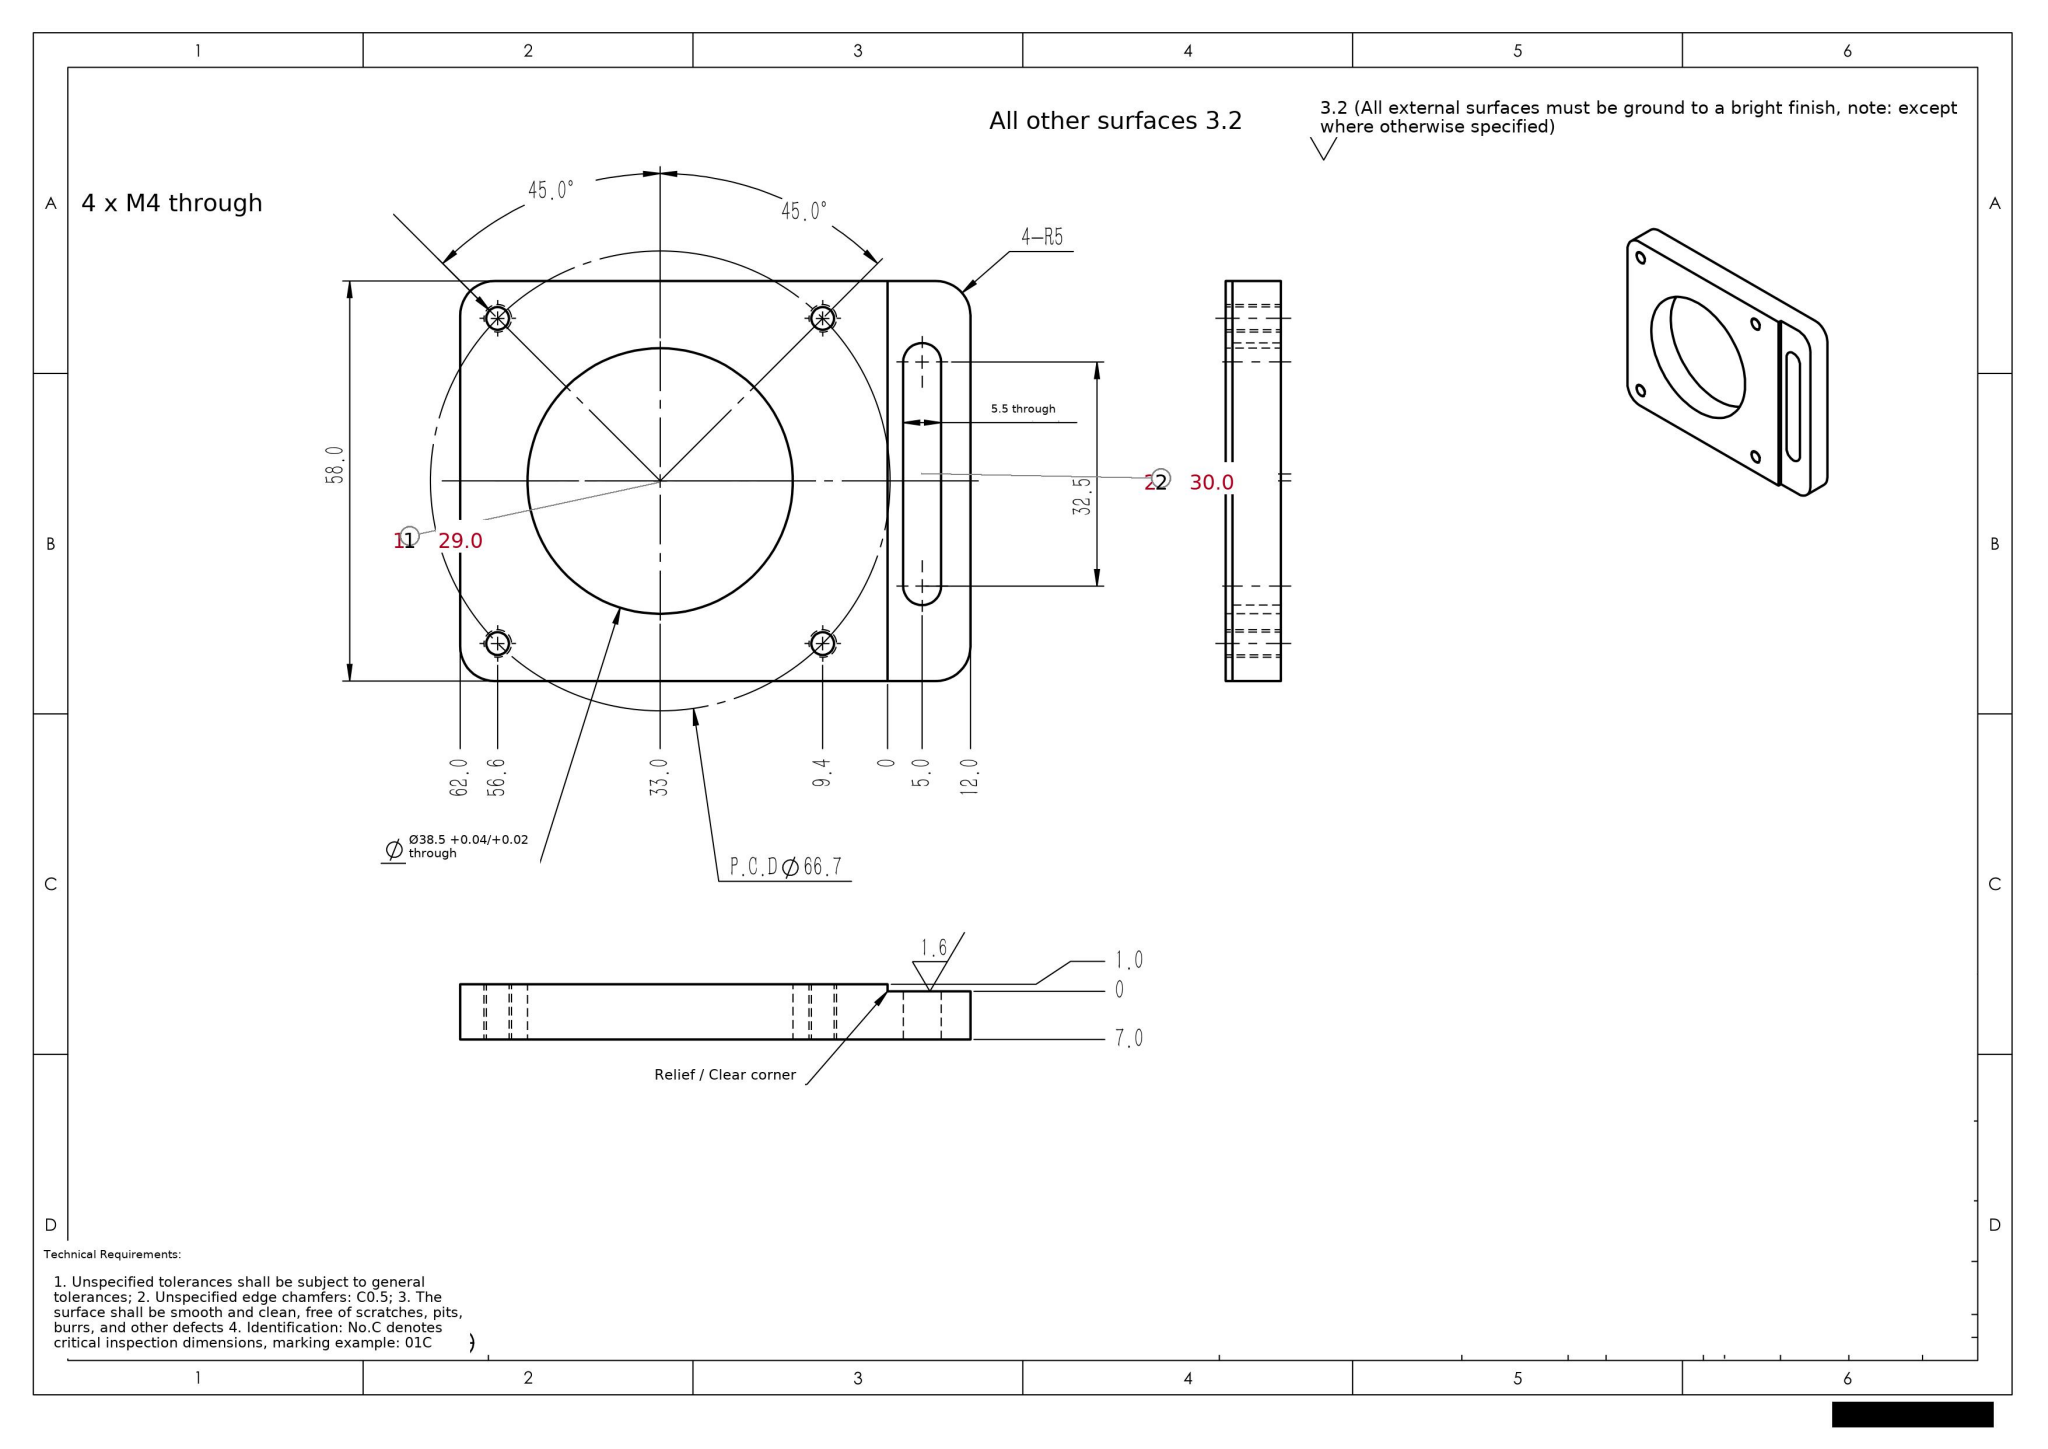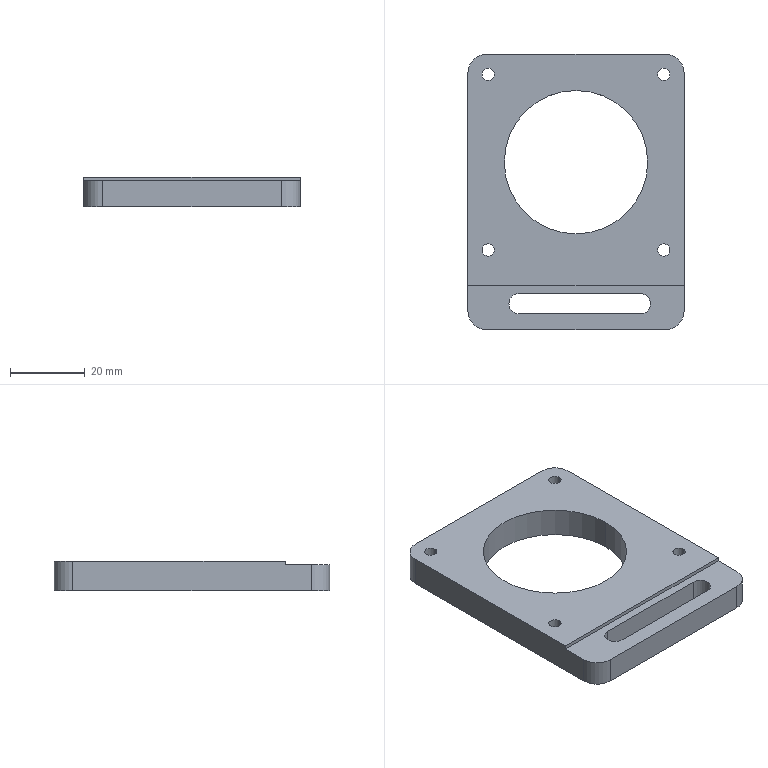Part | SolidWorks | mm | 1 solid | 27 faces | box 58 x 74 x 8 mm | volume 22475 mm3 | cylinder 17 | plane 10 | commonest cylinder face diameters 3.3 x8 10 x4 5.5 x3 38.5 x2
STEP:
#1=CARTESIAN_POINT('',(21.92,-15.57,0.));
#2=VERTEX_POINT('',#1);
#3=CARTESIAN_POINT('',(25.22,-15.57,0.));
#4=VERTEX_POINT('',#3);
#5=CARTESIAN_POINT('',(23.57,-15.57,0.));
#6=DIRECTION('',(0.,0.,1.));
#7=DIRECTION('',(1.,0.,0.));
#8=AXIS2_PLACEMENT_3D('',#5,#6,#7);
#9=CIRCLE('',#8,1.65);
#10=EDGE_CURVE('',#2,#4,#9,.T.);
#11=ORIENTED_EDGE('',*,*,#10,.F.);
#12=CARTESIAN_POINT('',(21.92,-15.57,8.));
#13=VERTEX_POINT('',#12);
#14=CARTESIAN_POINT('',(21.92,-15.57,8.));
#15=DIRECTION('',(0.,0.,1.));
#16=VECTOR('',#15,1000.);
#17=LINE('',#14,#16);
#18=EDGE_CURVE('',#2,#13,#17,.T.);
#19=ORIENTED_EDGE('',*,*,#18,.T.);
#20=CARTESIAN_POINT('',(25.22,-15.57,8.));
#21=VERTEX_POINT('',#20);
#22=CARTESIAN_POINT('',(23.57,-15.57,8.));
#23=DIRECTION('',(0.,0.,1.));
#24=DIRECTION('',(1.,0.,0.));
#25=AXIS2_PLACEMENT_3D('',#22,#23,#24);
#26=CIRCLE('',#25,1.65);
#27=EDGE_CURVE('',#13,#21,#26,.T.);
#28=ORIENTED_EDGE('',*,*,#27,.T.);
#29=CARTESIAN_POINT('',(25.22,-15.57,8.));
#30=DIRECTION('',(0.,0.,1.));
#31=VECTOR('',#30,1000.);
#32=LINE('',#29,#31);
#33=EDGE_CURVE('',#4,#21,#32,.T.);
#34=ORIENTED_EDGE('',*,*,#33,.F.);
#35=EDGE_LOOP('',(#11,#19,#28,#34));
#36=FACE_OUTER_BOUND('',#35,.T.);
#37=CARTESIAN_POINT('',(23.57,-15.57,8.));
#38=DIRECTION('',(0.,0.,1.));
#39=DIRECTION('',(1.,0.,0.));
#40=AXIS2_PLACEMENT_3D('',#37,#38,#39);
#41=CYLINDRICAL_SURFACE('',#40,1.65);
#42=ADVANCED_FACE('',(#36),#41,.F.);
#43=CARTESIAN_POINT('',(-25.22,-15.57,0.));
#44=VERTEX_POINT('',#43);
#45=CARTESIAN_POINT('',(-21.92,-15.57,0.));
#46=VERTEX_POINT('',#45);
#47=CARTESIAN_POINT('',(-23.57,-15.57,0.));
#48=DIRECTION('',(0.,0.,1.));
#49=DIRECTION('',(1.,0.,0.));
#50=AXIS2_PLACEMENT_3D('',#47,#48,#49);
#51=CIRCLE('',#50,1.65);
#52=EDGE_CURVE('',#44,#46,#51,.T.);
#53=ORIENTED_EDGE('',*,*,#52,.F.);
#54=CARTESIAN_POINT('',(-25.22,-15.57,8.));
#55=VERTEX_POINT('',#54);
#56=CARTESIAN_POINT('',(-25.22,-15.57,8.));
#57=DIRECTION('',(0.,0.,1.));
#58=VECTOR('',#57,1000.);
#59=LINE('',#56,#58);
#60=EDGE_CURVE('',#44,#55,#59,.T.);
#61=ORIENTED_EDGE('',*,*,#60,.T.);
#62=CARTESIAN_POINT('',(-21.92,-15.57,8.));
#63=VERTEX_POINT('',#62);
#64=CARTESIAN_POINT('',(-23.57,-15.57,8.));
#65=DIRECTION('',(0.,0.,1.));
#66=DIRECTION('',(1.,0.,0.));
#67=AXIS2_PLACEMENT_3D('',#64,#65,#66);
#68=CIRCLE('',#67,1.65);
#69=EDGE_CURVE('',#55,#63,#68,.T.);
#70=ORIENTED_EDGE('',*,*,#69,.T.);
#71=CARTESIAN_POINT('',(-21.92,-15.57,8.));
#72=DIRECTION('',(0.,0.,1.));
#73=VECTOR('',#72,1000.);
#74=LINE('',#71,#73);
#75=EDGE_CURVE('',#46,#63,#74,.T.);
#76=ORIENTED_EDGE('',*,*,#75,.F.);
#77=EDGE_LOOP('',(#53,#61,#70,#76));
#78=FACE_OUTER_BOUND('',#77,.T.);
#79=CARTESIAN_POINT('',(-23.57,-15.57,8.));
#80=DIRECTION('',(0.,0.,1.));
#81=DIRECTION('',(1.,0.,0.));
#82=AXIS2_PLACEMENT_3D('',#79,#80,#81);
#83=CYLINDRICAL_SURFACE('',#82,1.65);
#84=ADVANCED_FACE('',(#78),#83,.F.);
#85=CARTESIAN_POINT('',(-25.22,31.57,0.));
#86=VERTEX_POINT('',#85);
#87=CARTESIAN_POINT('',(-21.92,31.57,0.));
#88=VERTEX_POINT('',#87);
#89=CARTESIAN_POINT('',(-23.57,31.57,0.));
#90=DIRECTION('',(0.,0.,1.));
#91=DIRECTION('',(1.,0.,0.));
#92=AXIS2_PLACEMENT_3D('',#89,#90,#91);
#93=CIRCLE('',#92,1.65);
#94=EDGE_CURVE('',#86,#88,#93,.T.);
#95=ORIENTED_EDGE('',*,*,#94,.F.);
#96=CARTESIAN_POINT('',(-25.22,31.57,8.));
#97=VERTEX_POINT('',#96);
#98=CARTESIAN_POINT('',(-25.22,31.57,8.));
#99=DIRECTION('',(0.,0.,1.));
#100=VECTOR('',#99,1000.);
#101=LINE('',#98,#100);
#102=EDGE_CURVE('',#86,#97,#101,.T.);
#103=ORIENTED_EDGE('',*,*,#102,.T.);
#104=CARTESIAN_POINT('',(-21.92,31.57,8.));
#105=VERTEX_POINT('',#104);
#106=CARTESIAN_POINT('',(-23.57,31.57,8.));
#107=DIRECTION('',(0.,0.,1.));
#108=DIRECTION('',(1.,0.,0.));
#109=AXIS2_PLACEMENT_3D('',#106,#107,#108);
#110=CIRCLE('',#109,1.65);
#111=EDGE_CURVE('',#97,#105,#110,.T.);
#112=ORIENTED_EDGE('',*,*,#111,.T.);
#113=CARTESIAN_POINT('',(-21.92,31.57,8.));
#114=DIRECTION('',(0.,0.,1.));
#115=VECTOR('',#114,1000.);
#116=LINE('',#113,#115);
#117=EDGE_CURVE('',#88,#105,#116,.T.);
#118=ORIENTED_EDGE('',*,*,#117,.F.);
#119=EDGE_LOOP('',(#95,#103,#112,#118));
#120=FACE_OUTER_BOUND('',#119,.T.);
#121=CARTESIAN_POINT('',(-23.57,31.57,8.));
#122=DIRECTION('',(0.,0.,1.));
#123=DIRECTION('',(1.,0.,0.));
#124=AXIS2_PLACEMENT_3D('',#121,#122,#123);
#125=CYLINDRICAL_SURFACE('',#124,1.65);
#126=ADVANCED_FACE('',(#120),#125,.F.);
#127=CARTESIAN_POINT('',(21.92,31.57,0.));
#128=VERTEX_POINT('',#127);
#129=CARTESIAN_POINT('',(25.22,31.57,0.));
#130=VERTEX_POINT('',#129);
#131=CARTESIAN_POINT('',(23.57,31.57,0.));
#132=DIRECTION('',(0.,0.,1.));
#133=DIRECTION('',(1.,0.,0.));
#134=AXIS2_PLACEMENT_3D('',#131,#132,#133);
#135=CIRCLE('',#134,1.65);
#136=EDGE_CURVE('',#128,#130,#135,.T.);
#137=ORIENTED_EDGE('',*,*,#136,.F.);
#138=CARTESIAN_POINT('',(21.92,31.57,8.));
#139=VERTEX_POINT('',#138);
#140=CARTESIAN_POINT('',(21.92,31.57,8.));
#141=DIRECTION('',(0.,0.,1.));
#142=VECTOR('',#141,1000.);
#143=LINE('',#140,#142);
#144=EDGE_CURVE('',#128,#139,#143,.T.);
#145=ORIENTED_EDGE('',*,*,#144,.T.);
#146=CARTESIAN_POINT('',(25.22,31.57,8.));
#147=VERTEX_POINT('',#146);
#148=CARTESIAN_POINT('',(23.57,31.57,8.));
#149=DIRECTION('',(0.,0.,1.));
#150=DIRECTION('',(1.,0.,0.));
#151=AXIS2_PLACEMENT_3D('',#148,#149,#150);
#152=CIRCLE('',#151,1.65);
#153=EDGE_CURVE('',#139,#147,#152,.T.);
#154=ORIENTED_EDGE('',*,*,#153,.T.);
#155=CARTESIAN_POINT('',(25.22,31.57,8.));
#156=DIRECTION('',(0.,0.,1.));
#157=VECTOR('',#156,1000.);
#158=LINE('',#155,#157);
#159=EDGE_CURVE('',#130,#147,#158,.T.);
#160=ORIENTED_EDGE('',*,*,#159,.F.);
#161=EDGE_LOOP('',(#137,#145,#154,#160));
#162=FACE_OUTER_BOUND('',#161,.T.);
#163=CARTESIAN_POINT('',(23.57,31.57,8.));
#164=DIRECTION('',(0.,0.,1.));
#165=DIRECTION('',(1.,0.,0.));
#166=AXIS2_PLACEMENT_3D('',#163,#164,#165);
#167=CYLINDRICAL_SURFACE('',#166,1.65);
#168=ADVANCED_FACE('',(#162),#167,.F.);
#169=CARTESIAN_POINT('',(-15.25,-27.25,7.));
#170=VERTEX_POINT('',#169);
#171=CARTESIAN_POINT('',(-18.,-30.,7.));
#172=VERTEX_POINT('',#171);
#173=CARTESIAN_POINT('',(-15.25,-30.,7.));
#174=DIRECTION('',(0.,0.,1.));
#175=DIRECTION('',(1.,0.,0.));
#176=AXIS2_PLACEMENT_3D('',#173,#174,#175);
#177=CIRCLE('',#176,2.75);
#178=EDGE_CURVE('',#170,#172,#177,.T.);
#179=ORIENTED_EDGE('',*,*,#178,.T.);
#180=CARTESIAN_POINT('',(-18.,-30.,0.));
#181=VERTEX_POINT('',#180);
#182=CARTESIAN_POINT('',(-18.,-30.,0.));
#183=DIRECTION('',(0.,0.,-1.));
#184=VECTOR('',#183,1000.);
#185=LINE('',#182,#184);
#186=EDGE_CURVE('',#172,#181,#185,.T.);
#187=ORIENTED_EDGE('',*,*,#186,.T.);
#188=CARTESIAN_POINT('',(-15.25,-27.25,0.));
#189=VERTEX_POINT('',#188);
#190=CARTESIAN_POINT('',(-15.25,-30.,0.));
#191=DIRECTION('',(0.,0.,-1.));
#192=DIRECTION('',(-1.,0.,0.));
#193=AXIS2_PLACEMENT_3D('',#190,#191,#192);
#194=CIRCLE('',#193,2.75);
#195=EDGE_CURVE('',#181,#189,#194,.T.);
#196=ORIENTED_EDGE('',*,*,#195,.T.);
#197=CARTESIAN_POINT('',(-15.25,-27.25,0.));
#198=DIRECTION('',(0.,0.,-1.));
#199=VECTOR('',#198,1000.);
#200=LINE('',#197,#199);
#201=EDGE_CURVE('',#170,#189,#200,.T.);
#202=ORIENTED_EDGE('',*,*,#201,.F.);
#203=EDGE_LOOP('',(#179,#187,#196,#202));
#204=FACE_OUTER_BOUND('',#203,.T.);
#205=CARTESIAN_POINT('',(-15.25,-30.,0.));
#206=DIRECTION('',(0.,0.,-1.));
#207=DIRECTION('',(-1.,0.,0.));
#208=AXIS2_PLACEMENT_3D('',#205,#206,#207);
#209=CYLINDRICAL_SURFACE('',#208,2.75);
#210=ADVANCED_FACE('',(#204),#209,.F.);
#211=CARTESIAN_POINT('',(-19.25,8.,0.));
#212=VERTEX_POINT('',#211);
#213=CARTESIAN_POINT('',(19.25,8.,0.));
#214=VERTEX_POINT('',#213);
#215=CARTESIAN_POINT('',(0.,8.,0.));
#216=DIRECTION('',(0.,0.,1.));
#217=DIRECTION('',(1.,0.,0.));
#218=AXIS2_PLACEMENT_3D('',#215,#216,#217);
#219=CIRCLE('',#218,19.25);
#220=EDGE_CURVE('',#212,#214,#219,.T.);
#221=ORIENTED_EDGE('',*,*,#220,.F.);
#222=CARTESIAN_POINT('',(-19.25,8.,8.));
#223=VERTEX_POINT('',#222);
#224=CARTESIAN_POINT('',(-19.25,8.,0.));
#225=DIRECTION('',(0.,0.,1.));
#226=VECTOR('',#225,1000.);
#227=LINE('',#224,#226);
#228=EDGE_CURVE('',#212,#223,#227,.T.);
#229=ORIENTED_EDGE('',*,*,#228,.T.);
#230=CARTESIAN_POINT('',(19.25,8.,8.));
#231=VERTEX_POINT('',#230);
#232=CARTESIAN_POINT('',(0.,8.,8.));
#233=DIRECTION('',(0.,0.,1.));
#234=DIRECTION('',(1.,0.,0.));
#235=AXIS2_PLACEMENT_3D('',#232,#233,#234);
#236=CIRCLE('',#235,19.25);
#237=EDGE_CURVE('',#223,#231,#236,.T.);
#238=ORIENTED_EDGE('',*,*,#237,.T.);
#239=CARTESIAN_POINT('',(19.25,8.,0.));
#240=DIRECTION('',(0.,0.,1.));
#241=VECTOR('',#240,1000.);
#242=LINE('',#239,#241);
#243=EDGE_CURVE('',#214,#231,#242,.T.);
#244=ORIENTED_EDGE('',*,*,#243,.F.);
#245=EDGE_LOOP('',(#221,#229,#238,#244));
#246=FACE_OUTER_BOUND('',#245,.T.);
#247=CARTESIAN_POINT('',(0.,8.,0.));
#248=DIRECTION('',(0.,0.,1.));
#249=DIRECTION('',(1.,0.,0.));
#250=AXIS2_PLACEMENT_3D('',#247,#248,#249);
#251=CYLINDRICAL_SURFACE('',#250,19.25);
#252=ADVANCED_FACE('',(#246),#251,.F.);
#253=CARTESIAN_POINT('',(-23.57,-15.57,8.));
#254=DIRECTION('',(0.,0.,1.));
#255=DIRECTION('',(1.,0.,0.));
#256=AXIS2_PLACEMENT_3D('',#253,#254,#255);
#257=CIRCLE('',#256,1.65);
#258=EDGE_CURVE('',#63,#55,#257,.T.);
#259=ORIENTED_EDGE('',*,*,#258,.F.);
#260=ORIENTED_EDGE('',*,*,#69,.F.);
#261=EDGE_LOOP('',(#259,#260));
#262=FACE_BOUND('',#261,.T.);
#263=CARTESIAN_POINT('',(-23.57,31.57,8.));
#264=DIRECTION('',(0.,0.,1.));
#265=DIRECTION('',(1.,0.,0.));
#266=AXIS2_PLACEMENT_3D('',#263,#264,#265);
#267=CIRCLE('',#266,1.65);
#268=EDGE_CURVE('',#105,#97,#267,.T.);
#269=ORIENTED_EDGE('',*,*,#268,.F.);
#270=ORIENTED_EDGE('',*,*,#111,.F.);
#271=EDGE_LOOP('',(#269,#270));
#272=FACE_BOUND('',#271,.T.);
#273=CARTESIAN_POINT('',(23.57,31.57,8.));
#274=DIRECTION('',(0.,0.,1.));
#275=DIRECTION('',(1.,0.,0.));
#276=AXIS2_PLACEMENT_3D('',#273,#274,#275);
#277=CIRCLE('',#276,1.65);
#278=EDGE_CURVE('',#147,#139,#277,.T.);
#279=ORIENTED_EDGE('',*,*,#278,.F.);
#280=ORIENTED_EDGE('',*,*,#153,.F.);
#281=EDGE_LOOP('',(#279,#280));
#282=FACE_BOUND('',#281,.T.);
#283=CARTESIAN_POINT('',(0.,8.,8.));
#284=DIRECTION('',(0.,0.,1.));
#285=DIRECTION('',(1.,0.,0.));
#286=AXIS2_PLACEMENT_3D('',#283,#284,#285);
#287=CIRCLE('',#286,19.25);
#288=EDGE_CURVE('',#231,#223,#287,.T.);
#289=ORIENTED_EDGE('',*,*,#288,.F.);
#290=ORIENTED_EDGE('',*,*,#237,.F.);
#291=EDGE_LOOP('',(#289,#290));
#292=FACE_BOUND('',#291,.T.);
#293=CARTESIAN_POINT('',(24.,37.,8.));
#294=VERTEX_POINT('',#293);
#295=CARTESIAN_POINT('',(-24.,37.,8.));
#296=VERTEX_POINT('',#295);
#297=CARTESIAN_POINT('',(29.,37.,8.));
#298=DIRECTION('',(-1.,-0.,0.));
#299=VECTOR('',#298,1000.);
#300=LINE('',#297,#299);
#301=EDGE_CURVE('',#294,#296,#300,.T.);
#302=ORIENTED_EDGE('',*,*,#301,.T.);
#303=CARTESIAN_POINT('',(-29.,32.,8.));
#304=VERTEX_POINT('',#303);
#305=CARTESIAN_POINT('',(-24.,32.,8.));
#306=DIRECTION('',(0.,0.,1.));
#307=DIRECTION('',(-1.,0.,0.));
#308=AXIS2_PLACEMENT_3D('',#305,#306,#307);
#309=CIRCLE('',#308,5.);
#310=EDGE_CURVE('',#296,#304,#309,.T.);
#311=ORIENTED_EDGE('',*,*,#310,.T.);
#312=CARTESIAN_POINT('',(-29.,-25.,8.));
#313=VERTEX_POINT('',#312);
#314=CARTESIAN_POINT('',(-29.,37.,8.));
#315=DIRECTION('',(0.,-1.,0.));
#316=VECTOR('',#315,1000.);
#317=LINE('',#314,#316);
#318=EDGE_CURVE('',#304,#313,#317,.T.);
#319=ORIENTED_EDGE('',*,*,#318,.T.);
#320=CARTESIAN_POINT('',(29.,-25.,8.));
#321=VERTEX_POINT('',#320);
#322=CARTESIAN_POINT('',(29.,-25.,8.));
#323=DIRECTION('',(-1.,-0.,0.));
#324=VECTOR('',#323,1000.);
#325=LINE('',#322,#324);
#326=EDGE_CURVE('',#321,#313,#325,.T.);
#327=ORIENTED_EDGE('',*,*,#326,.F.);
#328=CARTESIAN_POINT('',(29.,32.,8.));
#329=VERTEX_POINT('',#328);
#330=CARTESIAN_POINT('',(29.,37.,8.));
#331=DIRECTION('',(-0.,1.,0.));
#332=VECTOR('',#331,1000.);
#333=LINE('',#330,#332);
#334=EDGE_CURVE('',#321,#329,#333,.T.);
#335=ORIENTED_EDGE('',*,*,#334,.T.);
#336=CARTESIAN_POINT('',(24.,32.,8.));
#337=DIRECTION('',(0.,0.,1.));
#338=DIRECTION('',(-1.,0.,0.));
#339=AXIS2_PLACEMENT_3D('',#336,#337,#338);
#340=CIRCLE('',#339,5.);
#341=EDGE_CURVE('',#329,#294,#340,.T.);
#342=ORIENTED_EDGE('',*,*,#341,.T.);
#343=EDGE_LOOP('',(#302,#311,#319,#327,#335,#342));
#344=FACE_OUTER_BOUND('',#343,.T.);
#345=CARTESIAN_POINT('',(23.57,-15.57,8.));
#346=DIRECTION('',(0.,0.,1.));
#347=DIRECTION('',(1.,0.,0.));
#348=AXIS2_PLACEMENT_3D('',#345,#346,#347);
#349=CIRCLE('',#348,1.65);
#350=EDGE_CURVE('',#21,#13,#349,.T.);
#351=ORIENTED_EDGE('',*,*,#350,.F.);
#352=ORIENTED_EDGE('',*,*,#27,.F.);
#353=EDGE_LOOP('',(#351,#352));
#354=FACE_BOUND('',#353,.T.);
#355=CARTESIAN_POINT('',(0.,0.,8.));
#356=DIRECTION('',(0.,0.,-1.));
#357=DIRECTION('',(-1.,0.,0.));
#358=AXIS2_PLACEMENT_3D('',#355,#356,#357);
#359=PLANE('',#358);
#360=ADVANCED_FACE('',(#262,#272,#282,#292,#344,#354),#359,.F.);
#361=CARTESIAN_POINT('',(-24.,-37.,7.));
#362=VERTEX_POINT('',#361);
#363=CARTESIAN_POINT('',(24.,-37.,7.));
#364=VERTEX_POINT('',#363);
#365=CARTESIAN_POINT('',(29.,-37.,7.));
#366=DIRECTION('',(1.,0.,0.));
#367=VECTOR('',#366,1000.);
#368=LINE('',#365,#367);
#369=EDGE_CURVE('',#362,#364,#368,.T.);
#370=ORIENTED_EDGE('',*,*,#369,.F.);
#371=CARTESIAN_POINT('',(-24.,-37.,0.));
#372=VERTEX_POINT('',#371);
#373=CARTESIAN_POINT('',(-24.,-37.,8.));
#374=DIRECTION('',(0.,0.,-1.));
#375=VECTOR('',#374,1000.);
#376=LINE('',#373,#375);
#377=EDGE_CURVE('',#362,#372,#376,.T.);
#378=ORIENTED_EDGE('',*,*,#377,.T.);
#379=CARTESIAN_POINT('',(24.,-37.,0.));
#380=VERTEX_POINT('',#379);
#381=CARTESIAN_POINT('',(29.,-37.,0.));
#382=DIRECTION('',(1.,0.,0.));
#383=VECTOR('',#382,1000.);
#384=LINE('',#381,#383);
#385=EDGE_CURVE('',#372,#380,#384,.T.);
#386=ORIENTED_EDGE('',*,*,#385,.T.);
#387=CARTESIAN_POINT('',(24.,-37.,8.));
#388=DIRECTION('',(0.,0.,1.));
#389=VECTOR('',#388,1000.);
#390=LINE('',#387,#389);
#391=EDGE_CURVE('',#380,#364,#390,.T.);
#392=ORIENTED_EDGE('',*,*,#391,.T.);
#393=EDGE_LOOP('',(#370,#378,#386,#392));
#394=FACE_OUTER_BOUND('',#393,.T.);
#395=CARTESIAN_POINT('',(29.,-37.,8.));
#396=DIRECTION('',(-0.,1.,0.));
#397=DIRECTION('',(-1.,-0.,0.));
#398=AXIS2_PLACEMENT_3D('',#395,#396,#397);
#399=PLANE('',#398);
#400=ADVANCED_FACE('',(#394),#399,.F.);
#401=CARTESIAN_POINT('',(-29.,32.,0.));
#402=VERTEX_POINT('',#401);
#403=CARTESIAN_POINT('',(-29.,-32.,0.));
#404=VERTEX_POINT('',#403);
#405=CARTESIAN_POINT('',(-29.,37.,0.));
#406=DIRECTION('',(0.,-1.,0.));
#407=VECTOR('',#406,1000.);
#408=LINE('',#405,#407);
#409=EDGE_CURVE('',#402,#404,#408,.T.);
#410=ORIENTED_EDGE('',*,*,#409,.T.);
#411=CARTESIAN_POINT('',(-29.,-32.,7.));
#412=VERTEX_POINT('',#411);
#413=CARTESIAN_POINT('',(-29.,-32.,8.));
#414=DIRECTION('',(0.,0.,1.));
#415=VECTOR('',#414,1000.);
#416=LINE('',#413,#415);
#417=EDGE_CURVE('',#404,#412,#416,.T.);
#418=ORIENTED_EDGE('',*,*,#417,.T.);
#419=CARTESIAN_POINT('',(-29.,-25.,7.));
#420=VERTEX_POINT('',#419);
#421=CARTESIAN_POINT('',(-29.,-37.,7.));
#422=DIRECTION('',(-0.,-1.,0.));
#423=VECTOR('',#422,1000.);
#424=LINE('',#421,#423);
#425=EDGE_CURVE('',#420,#412,#424,.T.);
#426=ORIENTED_EDGE('',*,*,#425,.F.);
#427=CARTESIAN_POINT('',(-29.,-25.,7.));
#428=DIRECTION('',(0.,0.,1.));
#429=VECTOR('',#428,1000.);
#430=LINE('',#427,#429);
#431=EDGE_CURVE('',#420,#313,#430,.T.);
#432=ORIENTED_EDGE('',*,*,#431,.T.);
#433=ORIENTED_EDGE('',*,*,#318,.F.);
#434=CARTESIAN_POINT('',(-29.,32.,8.));
#435=DIRECTION('',(0.,0.,-1.));
#436=VECTOR('',#435,1000.);
#437=LINE('',#434,#436);
#438=EDGE_CURVE('',#304,#402,#437,.T.);
#439=ORIENTED_EDGE('',*,*,#438,.T.);
#440=EDGE_LOOP('',(#410,#418,#426,#432,#433,#439));
#441=FACE_OUTER_BOUND('',#440,.T.);
#442=CARTESIAN_POINT('',(-29.,37.,8.));
#443=DIRECTION('',(1.,0.,0.));
#444=DIRECTION('',(-0.,1.,0.));
#445=AXIS2_PLACEMENT_3D('',#442,#443,#444);
#446=PLANE('',#445);
#447=ADVANCED_FACE('',(#441),#446,.F.);
#448=CARTESIAN_POINT('',(29.,-32.,7.));
#449=VERTEX_POINT('',#448);
#450=CARTESIAN_POINT('',(29.,-25.,7.));
#451=VERTEX_POINT('',#450);
#452=CARTESIAN_POINT('',(29.,-37.,7.));
#453=DIRECTION('',(0.,1.,0.));
#454=VECTOR('',#453,1000.);
#455=LINE('',#452,#454);
#456=EDGE_CURVE('',#449,#451,#455,.T.);
#457=ORIENTED_EDGE('',*,*,#456,.F.);
#458=CARTESIAN_POINT('',(29.,-32.,0.));
#459=VERTEX_POINT('',#458);
#460=CARTESIAN_POINT('',(29.,-32.,8.));
#461=DIRECTION('',(0.,0.,-1.));
#462=VECTOR('',#461,1000.);
#463=LINE('',#460,#462);
#464=EDGE_CURVE('',#449,#459,#463,.T.);
#465=ORIENTED_EDGE('',*,*,#464,.T.);
#466=CARTESIAN_POINT('',(29.,32.,0.));
#467=VERTEX_POINT('',#466);
#468=CARTESIAN_POINT('',(29.,37.,0.));
#469=DIRECTION('',(-0.,1.,0.));
#470=VECTOR('',#469,1000.);
#471=LINE('',#468,#470);
#472=EDGE_CURVE('',#459,#467,#471,.T.);
#473=ORIENTED_EDGE('',*,*,#472,.T.);
#474=CARTESIAN_POINT('',(29.,32.,8.));
#475=DIRECTION('',(0.,0.,1.));
#476=VECTOR('',#475,1000.);
#477=LINE('',#474,#476);
#478=EDGE_CURVE('',#467,#329,#477,.T.);
#479=ORIENTED_EDGE('',*,*,#478,.T.);
#480=ORIENTED_EDGE('',*,*,#334,.F.);
#481=CARTESIAN_POINT('',(29.,-25.,7.));
#482=DIRECTION('',(0.,0.,1.));
#483=VECTOR('',#482,1000.);
#484=LINE('',#481,#483);
#485=EDGE_CURVE('',#451,#321,#484,.T.);
#486=ORIENTED_EDGE('',*,*,#485,.F.);
#487=EDGE_LOOP('',(#457,#465,#473,#479,#480,#486));
#488=FACE_OUTER_BOUND('',#487,.T.);
#489=CARTESIAN_POINT('',(29.,37.,8.));
#490=DIRECTION('',(-1.,-0.,0.));
#491=DIRECTION('',(0.,-1.,0.));
#492=AXIS2_PLACEMENT_3D('',#489,#490,#491);
#493=PLANE('',#492);
#494=ADVANCED_FACE('',(#488),#493,.F.);
#495=CARTESIAN_POINT('',(24.,37.,0.));
#496=VERTEX_POINT('',#495);
#497=CARTESIAN_POINT('',(-24.,37.,0.));
#498=VERTEX_POINT('',#497);
#499=CARTESIAN_POINT('',(29.,37.,0.));
#500=DIRECTION('',(-1.,-0.,0.));
#501=VECTOR('',#500,1000.);
#502=LINE('',#499,#501);
#503=EDGE_CURVE('',#496,#498,#502,.T.);
#504=ORIENTED_EDGE('',*,*,#503,.T.);
#505=CARTESIAN_POINT('',(-24.,37.,8.));
#506=DIRECTION('',(0.,0.,1.));
#507=VECTOR('',#506,1000.);
#508=LINE('',#505,#507);
#509=EDGE_CURVE('',#498,#296,#508,.T.);
#510=ORIENTED_EDGE('',*,*,#509,.T.);
#511=ORIENTED_EDGE('',*,*,#301,.F.);
#512=CARTESIAN_POINT('',(24.,37.,8.));
#513=DIRECTION('',(0.,0.,-1.));
#514=VECTOR('',#513,1000.);
#515=LINE('',#512,#514);
#516=EDGE_CURVE('',#294,#496,#515,.T.);
#517=ORIENTED_EDGE('',*,*,#516,.T.);
#518=EDGE_LOOP('',(#504,#510,#511,#517));
#519=FACE_OUTER_BOUND('',#518,.T.);
#520=CARTESIAN_POINT('',(29.,37.,8.));
#521=DIRECTION('',(0.,-1.,0.));
#522=DIRECTION('',(1.,0.,0.));
#523=AXIS2_PLACEMENT_3D('',#520,#521,#522);
#524=PLANE('',#523);
#525=ADVANCED_FACE('',(#519),#524,.F.);
#526=CARTESIAN_POINT('',(23.57,-15.57,0.));
#527=DIRECTION('',(0.,0.,1.));
#528=DIRECTION('',(1.,0.,0.));
#529=AXIS2_PLACEMENT_3D('',#526,#527,#528);
#530=CIRCLE('',#529,1.65);
#531=EDGE_CURVE('',#4,#2,#530,.T.);
#532=ORIENTED_EDGE('',*,*,#531,.T.);
#533=ORIENTED_EDGE('',*,*,#10,.T.);
#534=EDGE_LOOP('',(#532,#533));
#535=FACE_BOUND('',#534,.T.);
#536=CARTESIAN_POINT('',(-23.57,-15.57,0.));
#537=DIRECTION('',(0.,0.,1.));
#538=DIRECTION('',(1.,0.,0.));
#539=AXIS2_PLACEMENT_3D('',#536,#537,#538);
#540=CIRCLE('',#539,1.65);
#541=EDGE_CURVE('',#46,#44,#540,.T.);
#542=ORIENTED_EDGE('',*,*,#541,.T.);
#543=ORIENTED_EDGE('',*,*,#52,.T.);
#544=EDGE_LOOP('',(#542,#543));
#545=FACE_BOUND('',#544,.T.);
#546=CARTESIAN_POINT('',(-23.57,31.57,0.));
#547=DIRECTION('',(0.,0.,1.));
#548=DIRECTION('',(1.,0.,0.));
#549=AXIS2_PLACEMENT_3D('',#546,#547,#548);
#550=CIRCLE('',#549,1.65);
#551=EDGE_CURVE('',#88,#86,#550,.T.);
#552=ORIENTED_EDGE('',*,*,#551,.T.);
#553=ORIENTED_EDGE('',*,*,#94,.T.);
#554=EDGE_LOOP('',(#552,#553));
#555=FACE_BOUND('',#554,.T.);
#556=CARTESIAN_POINT('',(23.57,31.57,0.));
#557=DIRECTION('',(0.,0.,1.));
#558=DIRECTION('',(1.,0.,0.));
#559=AXIS2_PLACEMENT_3D('',#556,#557,#558);
#560=CIRCLE('',#559,1.65);
#561=EDGE_CURVE('',#130,#128,#560,.T.);
#562=ORIENTED_EDGE('',*,*,#561,.T.);
#563=ORIENTED_EDGE('',*,*,#136,.T.);
#564=EDGE_LOOP('',(#562,#563));
#565=FACE_BOUND('',#564,.T.);
#566=CARTESIAN_POINT('',(17.25,-27.25,0.));
#567=VERTEX_POINT('',#566);
#568=CARTESIAN_POINT('',(17.25,-32.75,0.));
#569=VERTEX_POINT('',#568);
#570=CARTESIAN_POINT('',(17.25,-30.,0.));
#571=DIRECTION('',(0.,0.,-1.));
#572=DIRECTION('',(-1.,0.,0.));
#573=AXIS2_PLACEMENT_3D('',#570,#571,#572);
#574=CIRCLE('',#573,2.75);
#575=EDGE_CURVE('',#567,#569,#574,.T.);
#576=ORIENTED_EDGE('',*,*,#575,.F.);
#577=CARTESIAN_POINT('',(-15.25,-27.25,0.));
#578=DIRECTION('',(1.,0.,0.));
#579=VECTOR('',#578,1000.);
#580=LINE('',#577,#579);
#581=EDGE_CURVE('',#189,#567,#580,.T.);
#582=ORIENTED_EDGE('',*,*,#581,.F.);
#583=ORIENTED_EDGE('',*,*,#195,.F.);
#584=CARTESIAN_POINT('',(-15.25,-32.75,0.));
#585=VERTEX_POINT('',#584);
#586=CARTESIAN_POINT('',(-15.25,-30.,0.));
#587=DIRECTION('',(0.,0.,-1.));
#588=DIRECTION('',(-1.,0.,0.));
#589=AXIS2_PLACEMENT_3D('',#586,#587,#588);
#590=CIRCLE('',#589,2.75);
#591=EDGE_CURVE('',#585,#181,#590,.T.);
#592=ORIENTED_EDGE('',*,*,#591,.F.);
#593=CARTESIAN_POINT('',(-15.25,-32.75,0.));
#594=DIRECTION('',(1.,0.,0.));
#595=VECTOR('',#594,1000.);
#596=LINE('',#593,#595);
#597=EDGE_CURVE('',#585,#569,#596,.T.);
#598=ORIENTED_EDGE('',*,*,#597,.T.);
#599=EDGE_LOOP('',(#576,#582,#583,#592,#598));
#600=FACE_BOUND('',#599,.T.);
#601=CARTESIAN_POINT('',(0.,8.,0.));
#602=DIRECTION('',(0.,0.,1.));
#603=DIRECTION('',(1.,0.,0.));
#604=AXIS2_PLACEMENT_3D('',#601,#602,#603);
#605=CIRCLE('',#604,19.25);
#606=EDGE_CURVE('',#214,#212,#605,.T.);
#607=ORIENTED_EDGE('',*,*,#606,.T.);
#608=ORIENTED_EDGE('',*,*,#220,.T.);
#609=EDGE_LOOP('',(#607,#608));
#610=FACE_BOUND('',#609,.T.);
#611=ORIENTED_EDGE('',*,*,#385,.F.);
#612=CARTESIAN_POINT('',(-24.,-32.,0.));
#613=DIRECTION('',(0.,0.,-1.));
#614=DIRECTION('',(-1.,0.,0.));
#615=AXIS2_PLACEMENT_3D('',#612,#613,#614);
#616=CIRCLE('',#615,5.);
#617=EDGE_CURVE('',#372,#404,#616,.T.);
#618=ORIENTED_EDGE('',*,*,#617,.T.);
#619=ORIENTED_EDGE('',*,*,#409,.F.);
#620=CARTESIAN_POINT('',(-24.,32.,0.));
#621=DIRECTION('',(0.,0.,-1.));
#622=DIRECTION('',(-1.,0.,0.));
#623=AXIS2_PLACEMENT_3D('',#620,#621,#622);
#624=CIRCLE('',#623,5.);
#625=EDGE_CURVE('',#402,#498,#624,.T.);
#626=ORIENTED_EDGE('',*,*,#625,.T.);
#627=ORIENTED_EDGE('',*,*,#503,.F.);
#628=CARTESIAN_POINT('',(24.,32.,0.));
#629=DIRECTION('',(0.,0.,-1.));
#630=DIRECTION('',(-1.,0.,0.));
#631=AXIS2_PLACEMENT_3D('',#628,#629,#630);
#632=CIRCLE('',#631,5.);
#633=EDGE_CURVE('',#496,#467,#632,.T.);
#634=ORIENTED_EDGE('',*,*,#633,.T.);
#635=ORIENTED_EDGE('',*,*,#472,.F.);
#636=CARTESIAN_POINT('',(24.,-32.,0.));
#637=DIRECTION('',(0.,0.,-1.));
#638=DIRECTION('',(-1.,0.,0.));
#639=AXIS2_PLACEMENT_3D('',#636,#637,#638);
#640=CIRCLE('',#639,5.);
#641=EDGE_CURVE('',#459,#380,#640,.T.);
#642=ORIENTED_EDGE('',*,*,#641,.T.);
#643=EDGE_LOOP('',(#611,#618,#619,#626,#627,#634,#635,#642));
#644=FACE_OUTER_BOUND('',#643,.T.);
#645=CARTESIAN_POINT('',(0.,0.,0.));
#646=DIRECTION('',(0.,0.,-1.));
#647=DIRECTION('',(-1.,0.,0.));
#648=AXIS2_PLACEMENT_3D('',#645,#646,#647);
#649=PLANE('',#648);
#650=ADVANCED_FACE('',(#535,#545,#555,#565,#600,#610,#644),#649,.T.);
#651=ORIENTED_EDGE('',*,*,#228,.F.);
#652=ORIENTED_EDGE('',*,*,#606,.F.);
#653=ORIENTED_EDGE('',*,*,#243,.T.);
#654=ORIENTED_EDGE('',*,*,#288,.T.);
#655=EDGE_LOOP('',(#651,#652,#653,#654));
#656=FACE_OUTER_BOUND('',#655,.T.);
#657=CARTESIAN_POINT('',(0.,8.,0.));
#658=DIRECTION('',(0.,0.,1.));
#659=DIRECTION('',(1.,0.,0.));
#660=AXIS2_PLACEMENT_3D('',#657,#658,#659);
#661=CYLINDRICAL_SURFACE('',#660,19.25);
#662=ADVANCED_FACE('',(#656),#661,.F.);
#663=ORIENTED_EDGE('',*,*,#326,.T.);
#664=ORIENTED_EDGE('',*,*,#431,.F.);
#665=CARTESIAN_POINT('',(29.,-25.,7.));
#666=DIRECTION('',(-1.,-0.,0.));
#667=VECTOR('',#666,1000.);
#668=LINE('',#665,#667);
#669=EDGE_CURVE('',#451,#420,#668,.T.);
#670=ORIENTED_EDGE('',*,*,#669,.F.);
#671=ORIENTED_EDGE('',*,*,#485,.T.);
#672=EDGE_LOOP('',(#663,#664,#670,#671));
#673=FACE_OUTER_BOUND('',#672,.T.);
#674=CARTESIAN_POINT('',(29.,-25.,7.));
#675=DIRECTION('',(-0.,1.,0.));
#676=DIRECTION('',(-1.,-0.,0.));
#677=AXIS2_PLACEMENT_3D('',#674,#675,#676);
#678=PLANE('',#677);
#679=ADVANCED_FACE('',(#673),#678,.F.);
#680=ORIENTED_EDGE('',*,*,#178,.F.);
#681=CARTESIAN_POINT('',(17.25,-27.25,7.));
#682=VERTEX_POINT('',#681);
#683=CARTESIAN_POINT('',(0.,-27.25,7.));
#684=DIRECTION('',(-1.,0.,0.));
#685=VECTOR('',#684,1000.);
#686=LINE('',#683,#685);
#687=EDGE_CURVE('',#682,#170,#686,.T.);
#688=ORIENTED_EDGE('',*,*,#687,.F.);
#689=CARTESIAN_POINT('',(17.25,-32.75,7.));
#690=VERTEX_POINT('',#689);
#691=CARTESIAN_POINT('',(17.25,-30.,7.));
#692=DIRECTION('',(0.,0.,1.));
#693=DIRECTION('',(1.,0.,0.));
#694=AXIS2_PLACEMENT_3D('',#691,#692,#693);
#695=CIRCLE('',#694,2.75);
#696=EDGE_CURVE('',#690,#682,#695,.T.);
#697=ORIENTED_EDGE('',*,*,#696,.F.);
#698=CARTESIAN_POINT('',(-15.25,-32.75,7.));
#699=VERTEX_POINT('',#698);
#700=CARTESIAN_POINT('',(0.,-32.75,7.));
#701=DIRECTION('',(1.,0.,0.));
#702=VECTOR('',#701,1000.);
#703=LINE('',#700,#702);
#704=EDGE_CURVE('',#699,#690,#703,.T.);
#705=ORIENTED_EDGE('',*,*,#704,.F.);
#706=CARTESIAN_POINT('',(-15.25,-30.,7.));
#707=DIRECTION('',(0.,0.,1.));
#708=DIRECTION('',(1.,0.,0.));
#709=AXIS2_PLACEMENT_3D('',#706,#707,#708);
#710=CIRCLE('',#709,2.75);
#711=EDGE_CURVE('',#172,#699,#710,.T.);
#712=ORIENTED_EDGE('',*,*,#711,.F.);
#713=EDGE_LOOP('',(#680,#688,#697,#705,#712));
#714=FACE_BOUND('',#713,.T.);
#715=ORIENTED_EDGE('',*,*,#425,.T.);
#716=CARTESIAN_POINT('',(-24.,-32.,7.));
#717=DIRECTION('',(0.,0.,1.));
#718=DIRECTION('',(1.,0.,0.));
#719=AXIS2_PLACEMENT_3D('',#716,#717,#718);
#720=CIRCLE('',#719,5.);
#721=EDGE_CURVE('',#412,#362,#720,.T.);
#722=ORIENTED_EDGE('',*,*,#721,.T.);
#723=ORIENTED_EDGE('',*,*,#369,.T.);
#724=CARTESIAN_POINT('',(24.,-32.,7.));
#725=DIRECTION('',(0.,0.,1.));
#726=DIRECTION('',(1.,0.,0.));
#727=AXIS2_PLACEMENT_3D('',#724,#725,#726);
#728=CIRCLE('',#727,5.);
#729=EDGE_CURVE('',#364,#449,#728,.T.);
#730=ORIENTED_EDGE('',*,*,#729,.T.);
#731=ORIENTED_EDGE('',*,*,#456,.T.);
#732=ORIENTED_EDGE('',*,*,#669,.T.);
#733=EDGE_LOOP('',(#715,#722,#723,#730,#731,#732));
#734=FACE_OUTER_BOUND('',#733,.T.);
#735=CARTESIAN_POINT('',(0.,0.,7.));
#736=DIRECTION('',(0.,0.,1.));
#737=DIRECTION('',(1.,0.,0.));
#738=AXIS2_PLACEMENT_3D('',#735,#736,#737);
#739=PLANE('',#738);
#740=ADVANCED_FACE('',(#714,#734),#739,.T.);
#741=ORIENTED_EDGE('',*,*,#721,.F.);
#742=ORIENTED_EDGE('',*,*,#417,.F.);
#743=ORIENTED_EDGE('',*,*,#617,.F.);
#744=ORIENTED_EDGE('',*,*,#377,.F.);
#745=EDGE_LOOP('',(#741,#742,#743,#744));
#746=FACE_OUTER_BOUND('',#745,.T.);
#747=CARTESIAN_POINT('',(-24.,-32.,8.));
#748=DIRECTION('',(0.,0.,-1.));
#749=DIRECTION('',(-1.,0.,0.));
#750=AXIS2_PLACEMENT_3D('',#747,#748,#749);
#751=CYLINDRICAL_SURFACE('',#750,5.);
#752=ADVANCED_FACE('',(#746),#751,.T.);
#753=ORIENTED_EDGE('',*,*,#729,.F.);
#754=ORIENTED_EDGE('',*,*,#391,.F.);
#755=ORIENTED_EDGE('',*,*,#641,.F.);
#756=ORIENTED_EDGE('',*,*,#464,.F.);
#757=EDGE_LOOP('',(#753,#754,#755,#756));
#758=FACE_OUTER_BOUND('',#757,.T.);
#759=CARTESIAN_POINT('',(24.,-32.,8.));
#760=DIRECTION('',(0.,0.,-1.));
#761=DIRECTION('',(-1.,0.,0.));
#762=AXIS2_PLACEMENT_3D('',#759,#760,#761);
#763=CYLINDRICAL_SURFACE('',#762,5.);
#764=ADVANCED_FACE('',(#758),#763,.T.);
#765=ORIENTED_EDGE('',*,*,#310,.F.);
#766=ORIENTED_EDGE('',*,*,#509,.F.);
#767=ORIENTED_EDGE('',*,*,#625,.F.);
#768=ORIENTED_EDGE('',*,*,#438,.F.);
#769=EDGE_LOOP('',(#765,#766,#767,#768));
#770=FACE_OUTER_BOUND('',#769,.T.);
#771=CARTESIAN_POINT('',(-24.,32.,8.));
#772=DIRECTION('',(0.,0.,-1.));
#773=DIRECTION('',(-1.,0.,0.));
#774=AXIS2_PLACEMENT_3D('',#771,#772,#773);
#775=CYLINDRICAL_SURFACE('',#774,5.);
#776=ADVANCED_FACE('',(#770),#775,.T.);
#777=ORIENTED_EDGE('',*,*,#341,.F.);
#778=ORIENTED_EDGE('',*,*,#478,.F.);
#779=ORIENTED_EDGE('',*,*,#633,.F.);
#780=ORIENTED_EDGE('',*,*,#516,.F.);
#781=EDGE_LOOP('',(#777,#778,#779,#780));
#782=FACE_OUTER_BOUND('',#781,.T.);
#783=CARTESIAN_POINT('',(24.,32.,8.));
#784=DIRECTION('',(0.,0.,-1.));
#785=DIRECTION('',(-1.,0.,0.));
#786=AXIS2_PLACEMENT_3D('',#783,#784,#785);
#787=CYLINDRICAL_SURFACE('',#786,5.);
#788=ADVANCED_FACE('',(#782),#787,.T.);
#789=ORIENTED_EDGE('',*,*,#696,.T.);
#790=CARTESIAN_POINT('',(17.25,-27.25,0.));
#791=DIRECTION('',(0.,0.,1.));
#792=VECTOR('',#791,1000.);
#793=LINE('',#790,#792);
#794=EDGE_CURVE('',#567,#682,#793,.T.);
#795=ORIENTED_EDGE('',*,*,#794,.F.);
#796=ORIENTED_EDGE('',*,*,#575,.T.);
#797=CARTESIAN_POINT('',(17.25,-32.75,0.));
#798=DIRECTION('',(0.,0.,-1.));
#799=VECTOR('',#798,1000.);
#800=LINE('',#797,#799);
#801=EDGE_CURVE('',#690,#569,#800,.T.);
#802=ORIENTED_EDGE('',*,*,#801,.F.);
#803=EDGE_LOOP('',(#789,#795,#796,#802));
#804=FACE_OUTER_BOUND('',#803,.T.);
#805=CARTESIAN_POINT('',(17.25,-30.,0.));
#806=DIRECTION('',(0.,0.,-1.));
#807=DIRECTION('',(-1.,0.,0.));
#808=AXIS2_PLACEMENT_3D('',#805,#806,#807);
#809=CYLINDRICAL_SURFACE('',#808,2.75);
#810=ADVANCED_FACE('',(#804),#809,.F.);
#811=ORIENTED_EDGE('',*,*,#186,.F.);
#812=ORIENTED_EDGE('',*,*,#711,.T.);
#813=CARTESIAN_POINT('',(-15.25,-32.75,0.));
#814=DIRECTION('',(0.,0.,1.));
#815=VECTOR('',#814,1000.);
#816=LINE('',#813,#815);
#817=EDGE_CURVE('',#585,#699,#816,.T.);
#818=ORIENTED_EDGE('',*,*,#817,.F.);
#819=ORIENTED_EDGE('',*,*,#591,.T.);
#820=EDGE_LOOP('',(#811,#812,#818,#819));
#821=FACE_OUTER_BOUND('',#820,.T.);
#822=CARTESIAN_POINT('',(-15.25,-30.,0.));
#823=DIRECTION('',(0.,0.,-1.));
#824=DIRECTION('',(-1.,0.,0.));
#825=AXIS2_PLACEMENT_3D('',#822,#823,#824);
#826=CYLINDRICAL_SURFACE('',#825,2.75);
#827=ADVANCED_FACE('',(#821),#826,.F.);
#828=ORIENTED_EDGE('',*,*,#704,.T.);
#829=ORIENTED_EDGE('',*,*,#801,.T.);
#830=ORIENTED_EDGE('',*,*,#597,.F.);
#831=ORIENTED_EDGE('',*,*,#817,.T.);
#832=EDGE_LOOP('',(#828,#829,#830,#831));
#833=FACE_OUTER_BOUND('',#832,.T.);
#834=CARTESIAN_POINT('',(-15.25,-32.75,0.));
#835=DIRECTION('',(0.,-1.,0.));
#836=DIRECTION('',(0.,0.,-1.));
#837=AXIS2_PLACEMENT_3D('',#834,#835,#836);
#838=PLANE('',#837);
#839=ADVANCED_FACE('',(#833),#838,.F.);
#840=ORIENTED_EDGE('',*,*,#687,.T.);
#841=ORIENTED_EDGE('',*,*,#201,.T.);
#842=ORIENTED_EDGE('',*,*,#581,.T.);
#843=ORIENTED_EDGE('',*,*,#794,.T.);
#844=EDGE_LOOP('',(#840,#841,#842,#843));
#845=FACE_OUTER_BOUND('',#844,.T.);
#846=CARTESIAN_POINT('',(-15.25,-27.25,0.));
#847=DIRECTION('',(0.,1.,0.));
#848=DIRECTION('',(0.,0.,1.));
#849=AXIS2_PLACEMENT_3D('',#846,#847,#848);
#850=PLANE('',#849);
#851=ADVANCED_FACE('',(#845),#850,.F.);
#852=ORIENTED_EDGE('',*,*,#144,.F.);
#853=ORIENTED_EDGE('',*,*,#561,.F.);
#854=ORIENTED_EDGE('',*,*,#159,.T.);
#855=ORIENTED_EDGE('',*,*,#278,.T.);
#856=EDGE_LOOP('',(#852,#853,#854,#855));
#857=FACE_OUTER_BOUND('',#856,.T.);
#858=CARTESIAN_POINT('',(23.57,31.57,8.));
#859=DIRECTION('',(0.,0.,1.));
#860=DIRECTION('',(1.,0.,0.));
#861=AXIS2_PLACEMENT_3D('',#858,#859,#860);
#862=CYLINDRICAL_SURFACE('',#861,1.65);
#863=ADVANCED_FACE('',(#857),#862,.F.);
#864=ORIENTED_EDGE('',*,*,#102,.F.);
#865=ORIENTED_EDGE('',*,*,#551,.F.);
#866=ORIENTED_EDGE('',*,*,#117,.T.);
#867=ORIENTED_EDGE('',*,*,#268,.T.);
#868=EDGE_LOOP('',(#864,#865,#866,#867));
#869=FACE_OUTER_BOUND('',#868,.T.);
#870=CARTESIAN_POINT('',(-23.57,31.57,8.));
#871=DIRECTION('',(0.,0.,1.));
#872=DIRECTION('',(1.,0.,0.));
#873=AXIS2_PLACEMENT_3D('',#870,#871,#872);
#874=CYLINDRICAL_SURFACE('',#873,1.65);
#875=ADVANCED_FACE('',(#869),#874,.F.);
#876=ORIENTED_EDGE('',*,*,#60,.F.);
#877=ORIENTED_EDGE('',*,*,#541,.F.);
#878=ORIENTED_EDGE('',*,*,#75,.T.);
#879=ORIENTED_EDGE('',*,*,#258,.T.);
#880=EDGE_LOOP('',(#876,#877,#878,#879));
#881=FACE_OUTER_BOUND('',#880,.T.);
#882=CARTESIAN_POINT('',(-23.57,-15.57,8.));
#883=DIRECTION('',(0.,0.,1.));
#884=DIRECTION('',(1.,0.,0.));
#885=AXIS2_PLACEMENT_3D('',#882,#883,#884);
#886=CYLINDRICAL_SURFACE('',#885,1.65);
#887=ADVANCED_FACE('',(#881),#886,.F.);
#888=ORIENTED_EDGE('',*,*,#18,.F.);
#889=ORIENTED_EDGE('',*,*,#531,.F.);
#890=ORIENTED_EDGE('',*,*,#33,.T.);
#891=ORIENTED_EDGE('',*,*,#350,.T.);
#892=EDGE_LOOP('',(#888,#889,#890,#891));
#893=FACE_OUTER_BOUND('',#892,.T.);
#894=CARTESIAN_POINT('',(23.57,-15.57,8.));
#895=DIRECTION('',(0.,0.,1.));
#896=DIRECTION('',(1.,0.,0.));
#897=AXIS2_PLACEMENT_3D('',#894,#895,#896);
#898=CYLINDRICAL_SURFACE('',#897,1.65);
#899=ADVANCED_FACE('',(#893),#898,.F.);
#900=CLOSED_SHELL('',(#42,#84,#126,#168,#210,#252,#360,#400,#447,#494,#525,#650,#662,#679,#740,#752,#764,#776,#788,#810,#827,#839,#851,#863,#875,#887,#899));
#901=MANIFOLD_SOLID_BREP('',#900);
#902=CARTESIAN_POINT('',(0.,0.,0.));
#903=DIRECTION('',(0.,0.,1.));
#904=DIRECTION('',(1.,0.,0.));
#905=AXIS2_PLACEMENT_3D('',#902,#903,#904);
#906=(LENGTH_UNIT()NAMED_UNIT(*)SI_UNIT(.MILLI.,.METRE.));
#907=UNCERTAINTY_MEASURE_WITH_UNIT(LENGTH_MEASURE(0.00001),#906,'','');
#908=(NAMED_UNIT(*)PLANE_ANGLE_UNIT()SI_UNIT($,.RADIAN.));
#909=(NAMED_UNIT(*)SI_UNIT($,.STERADIAN.)SOLID_ANGLE_UNIT());
#910=(GEOMETRIC_REPRESENTATION_CONTEXT(3)GLOBAL_UNCERTAINTY_ASSIGNED_CONTEXT((#907))GLOBAL_UNIT_ASSIGNED_CONTEXT((#906,#908,#909))REPRESENTATION_CONTEXT('',''));
#911=ADVANCED_BREP_SHAPE_REPRESENTATION('',(#901,#905),#910);